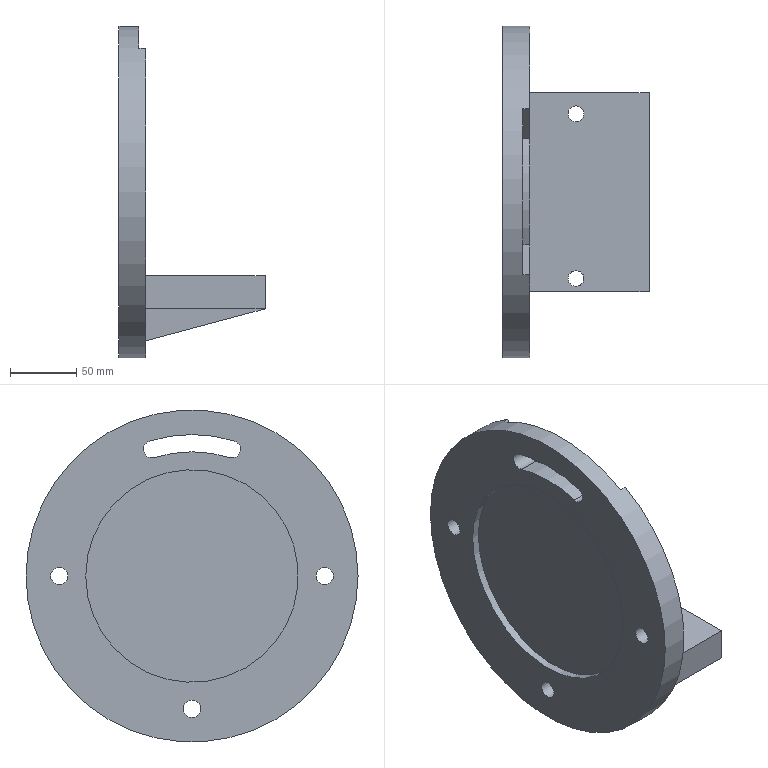Component | NX | FIXTURE_BODY | 1 solid | 39 faces | volume 1168497 mm3 | plane 19 | cylinder 16 | cone 4 | commonest cylinder face diameters 13 x5 3 x4 160 x2 12 x2 250 x1 187 x1 213 x1